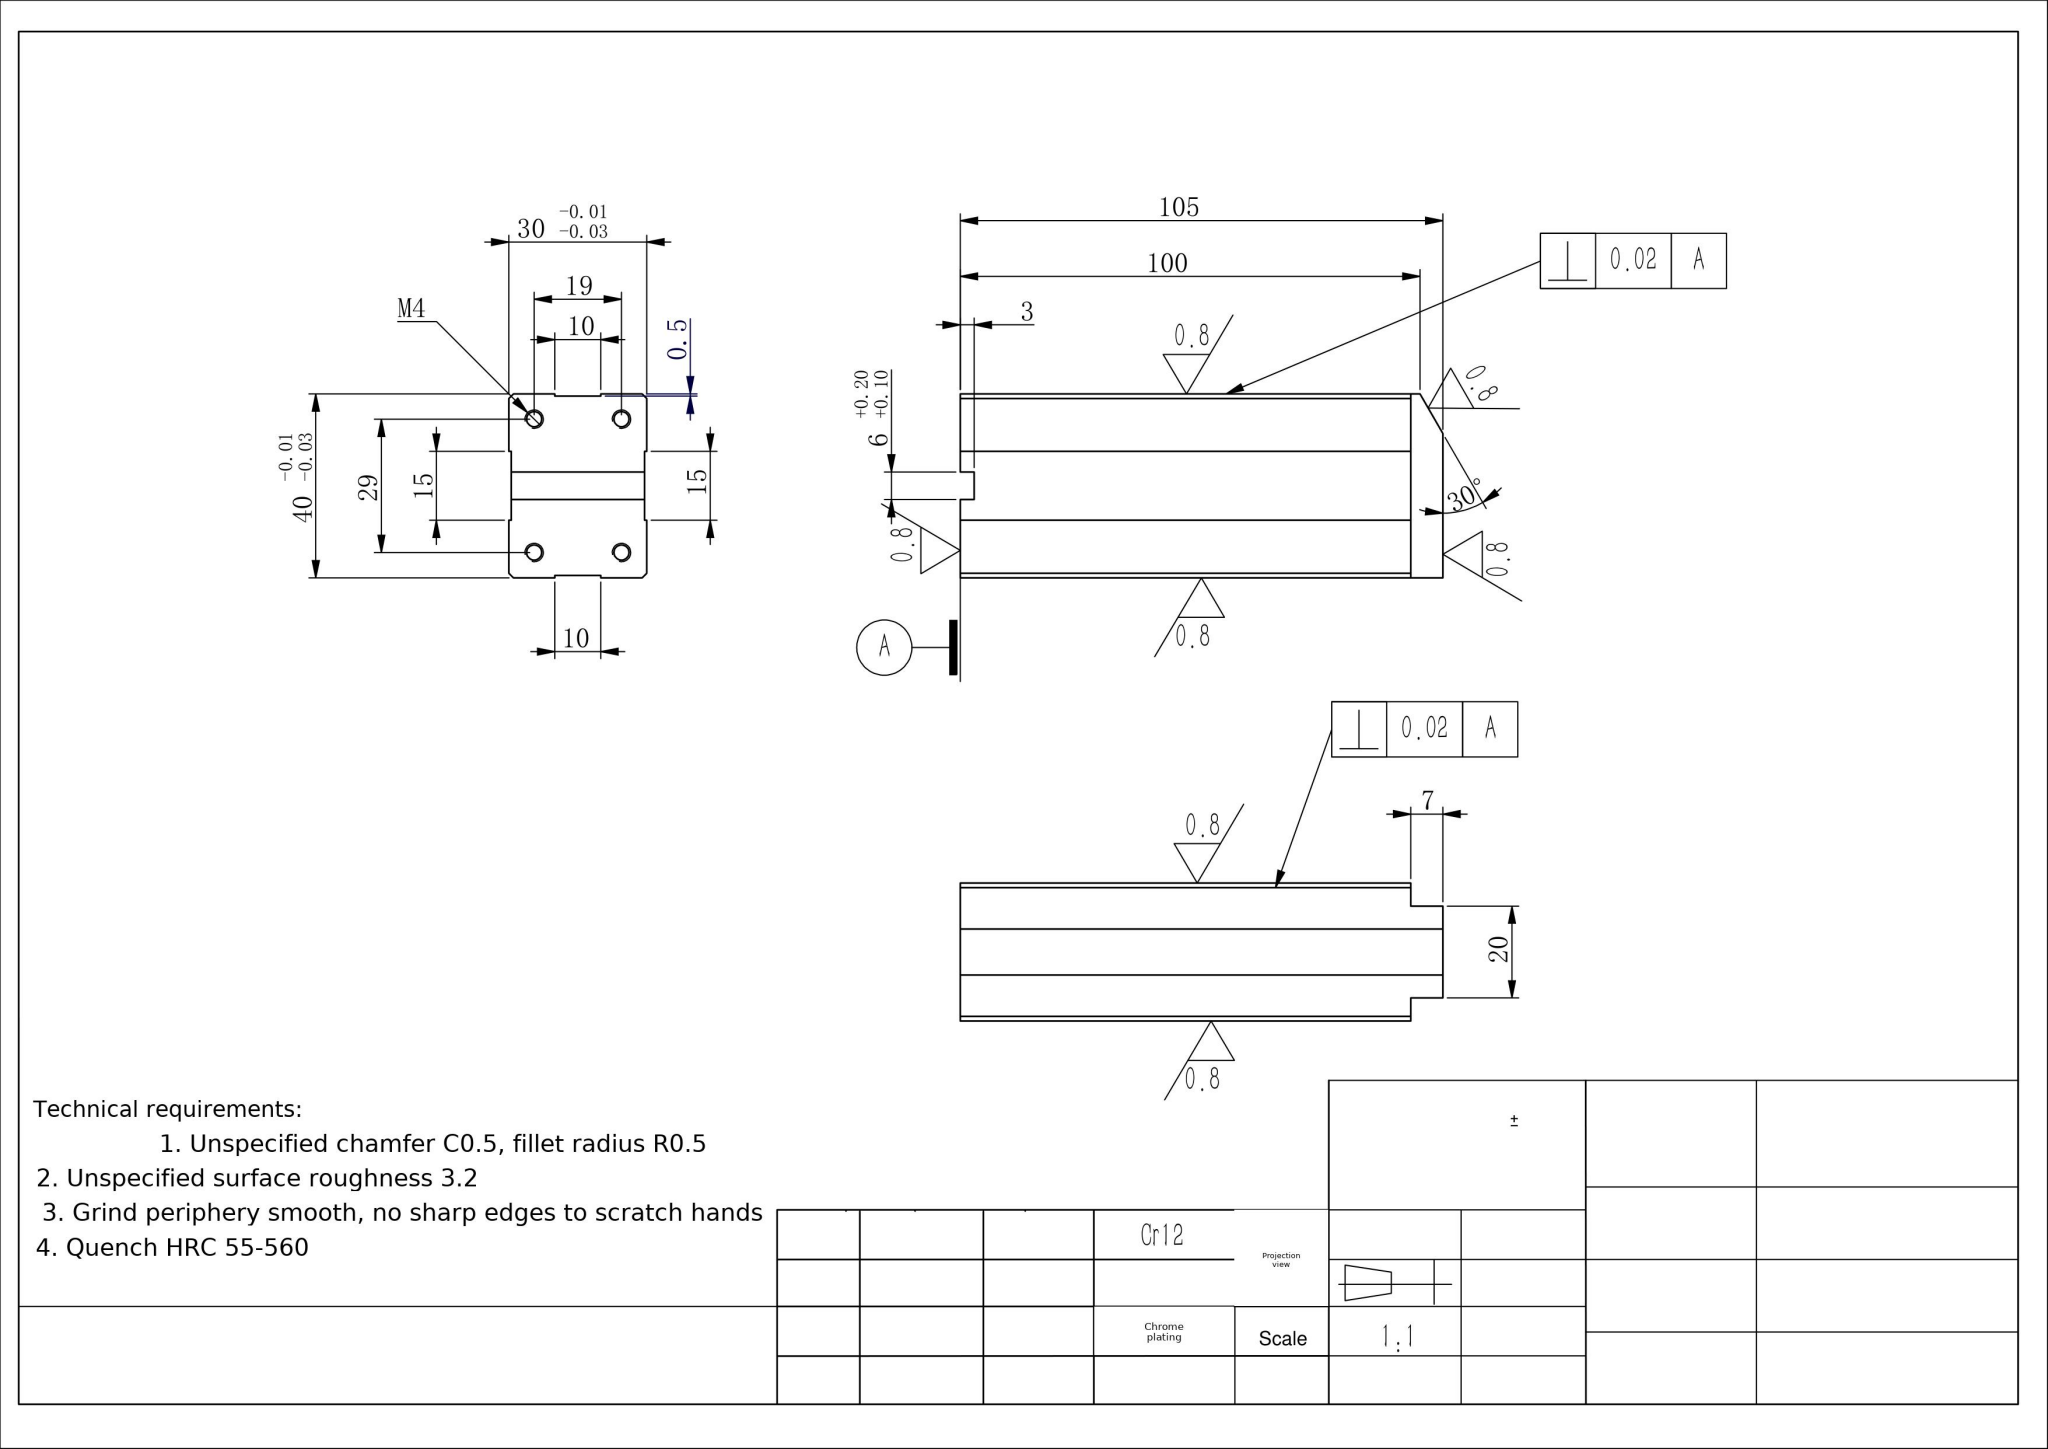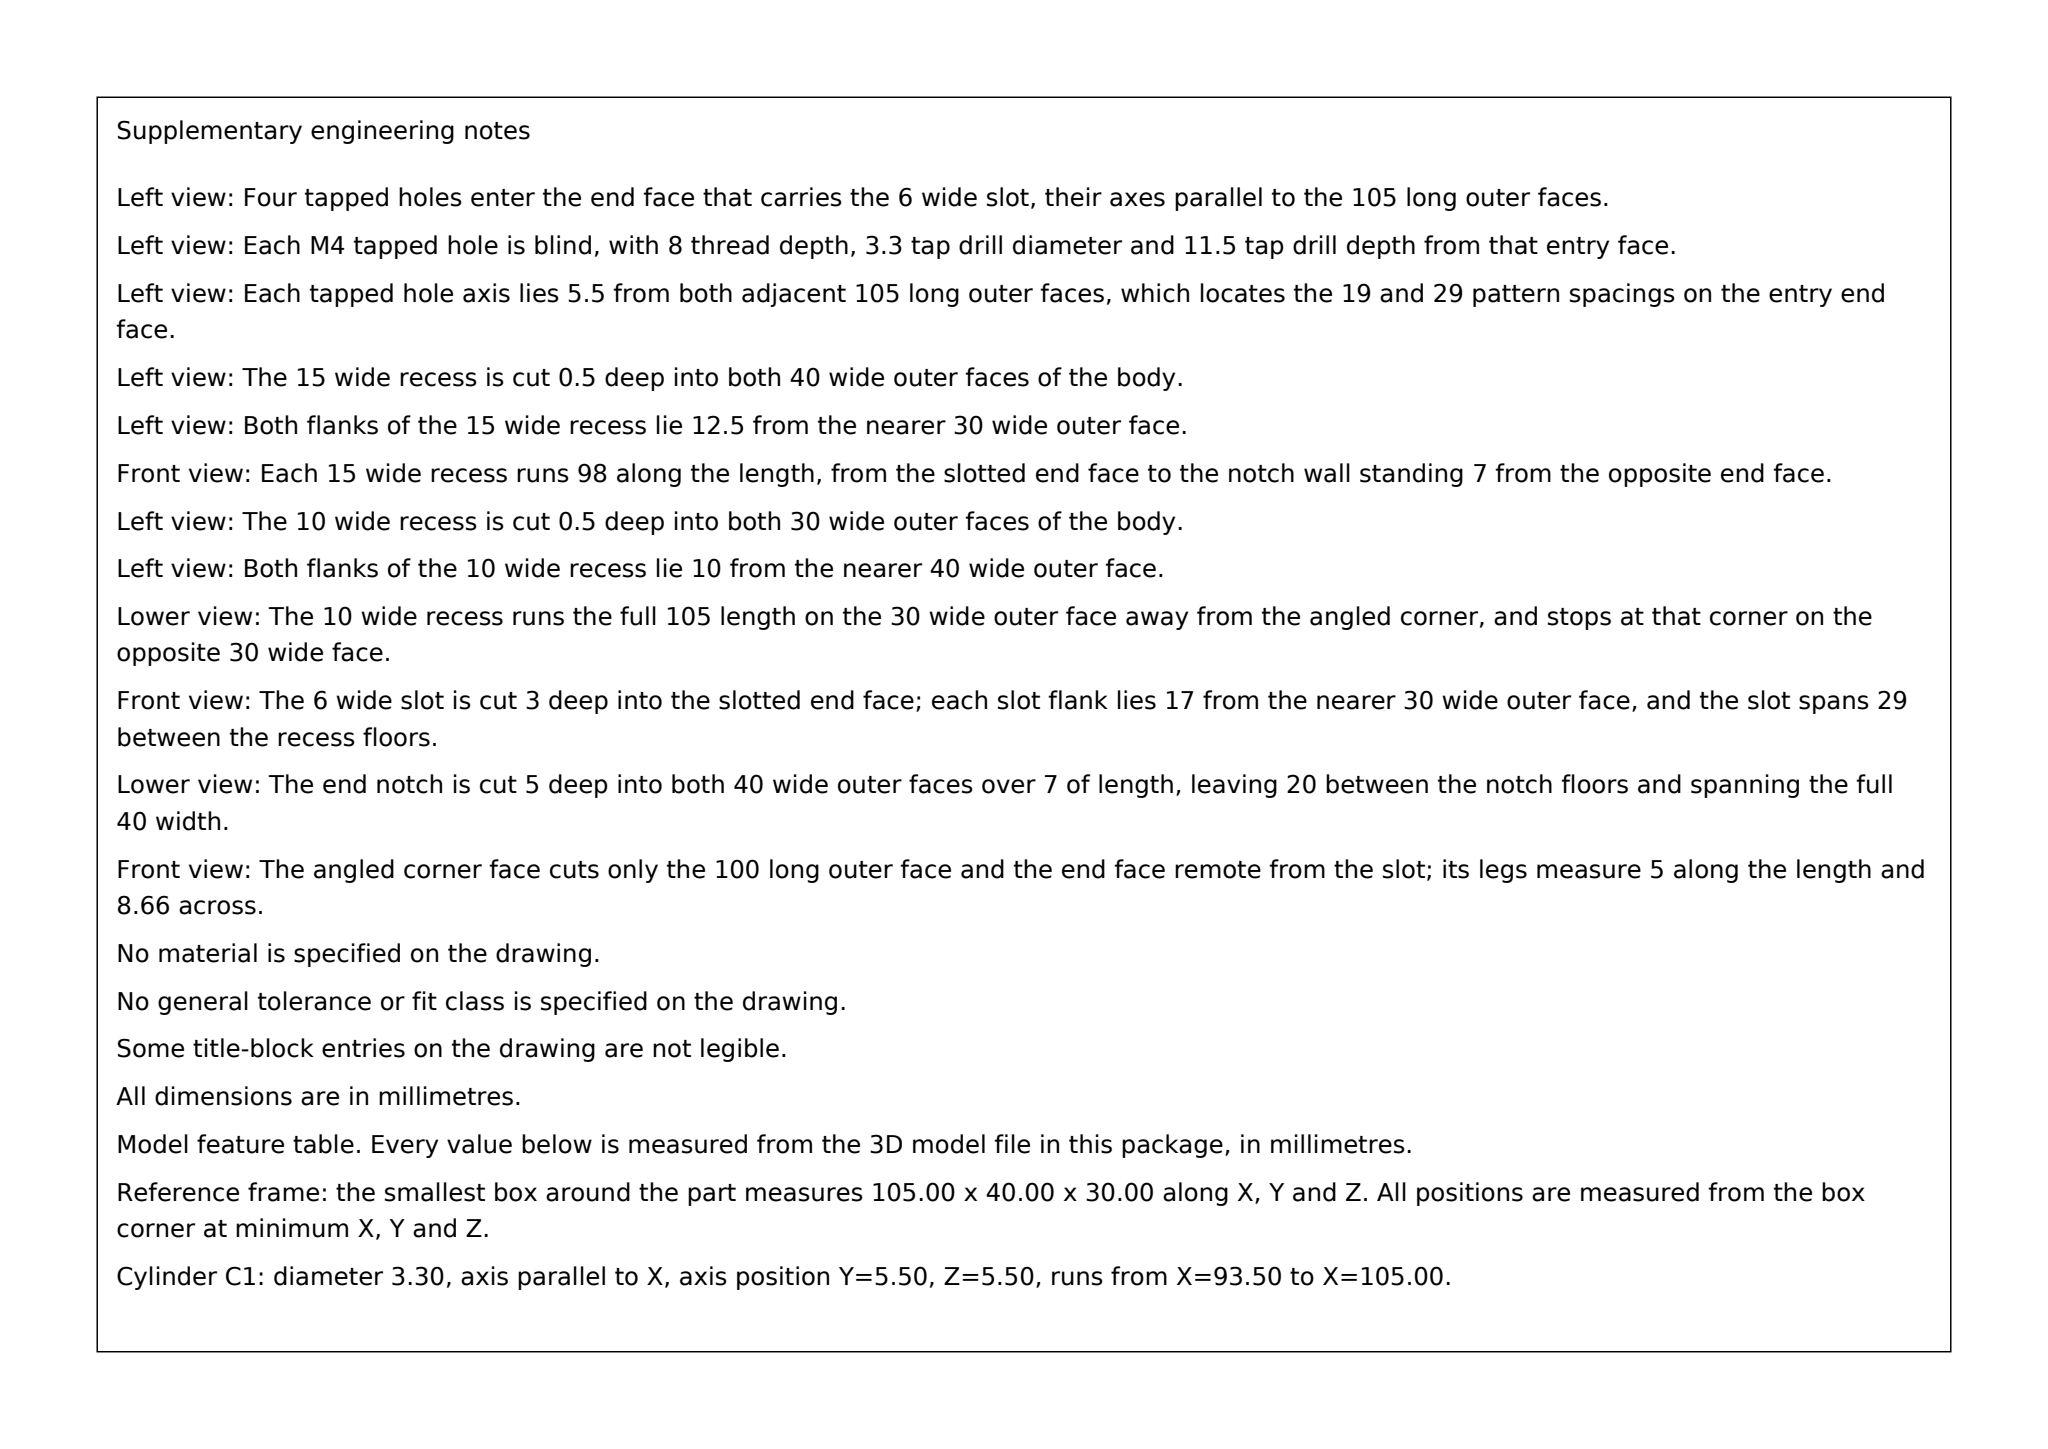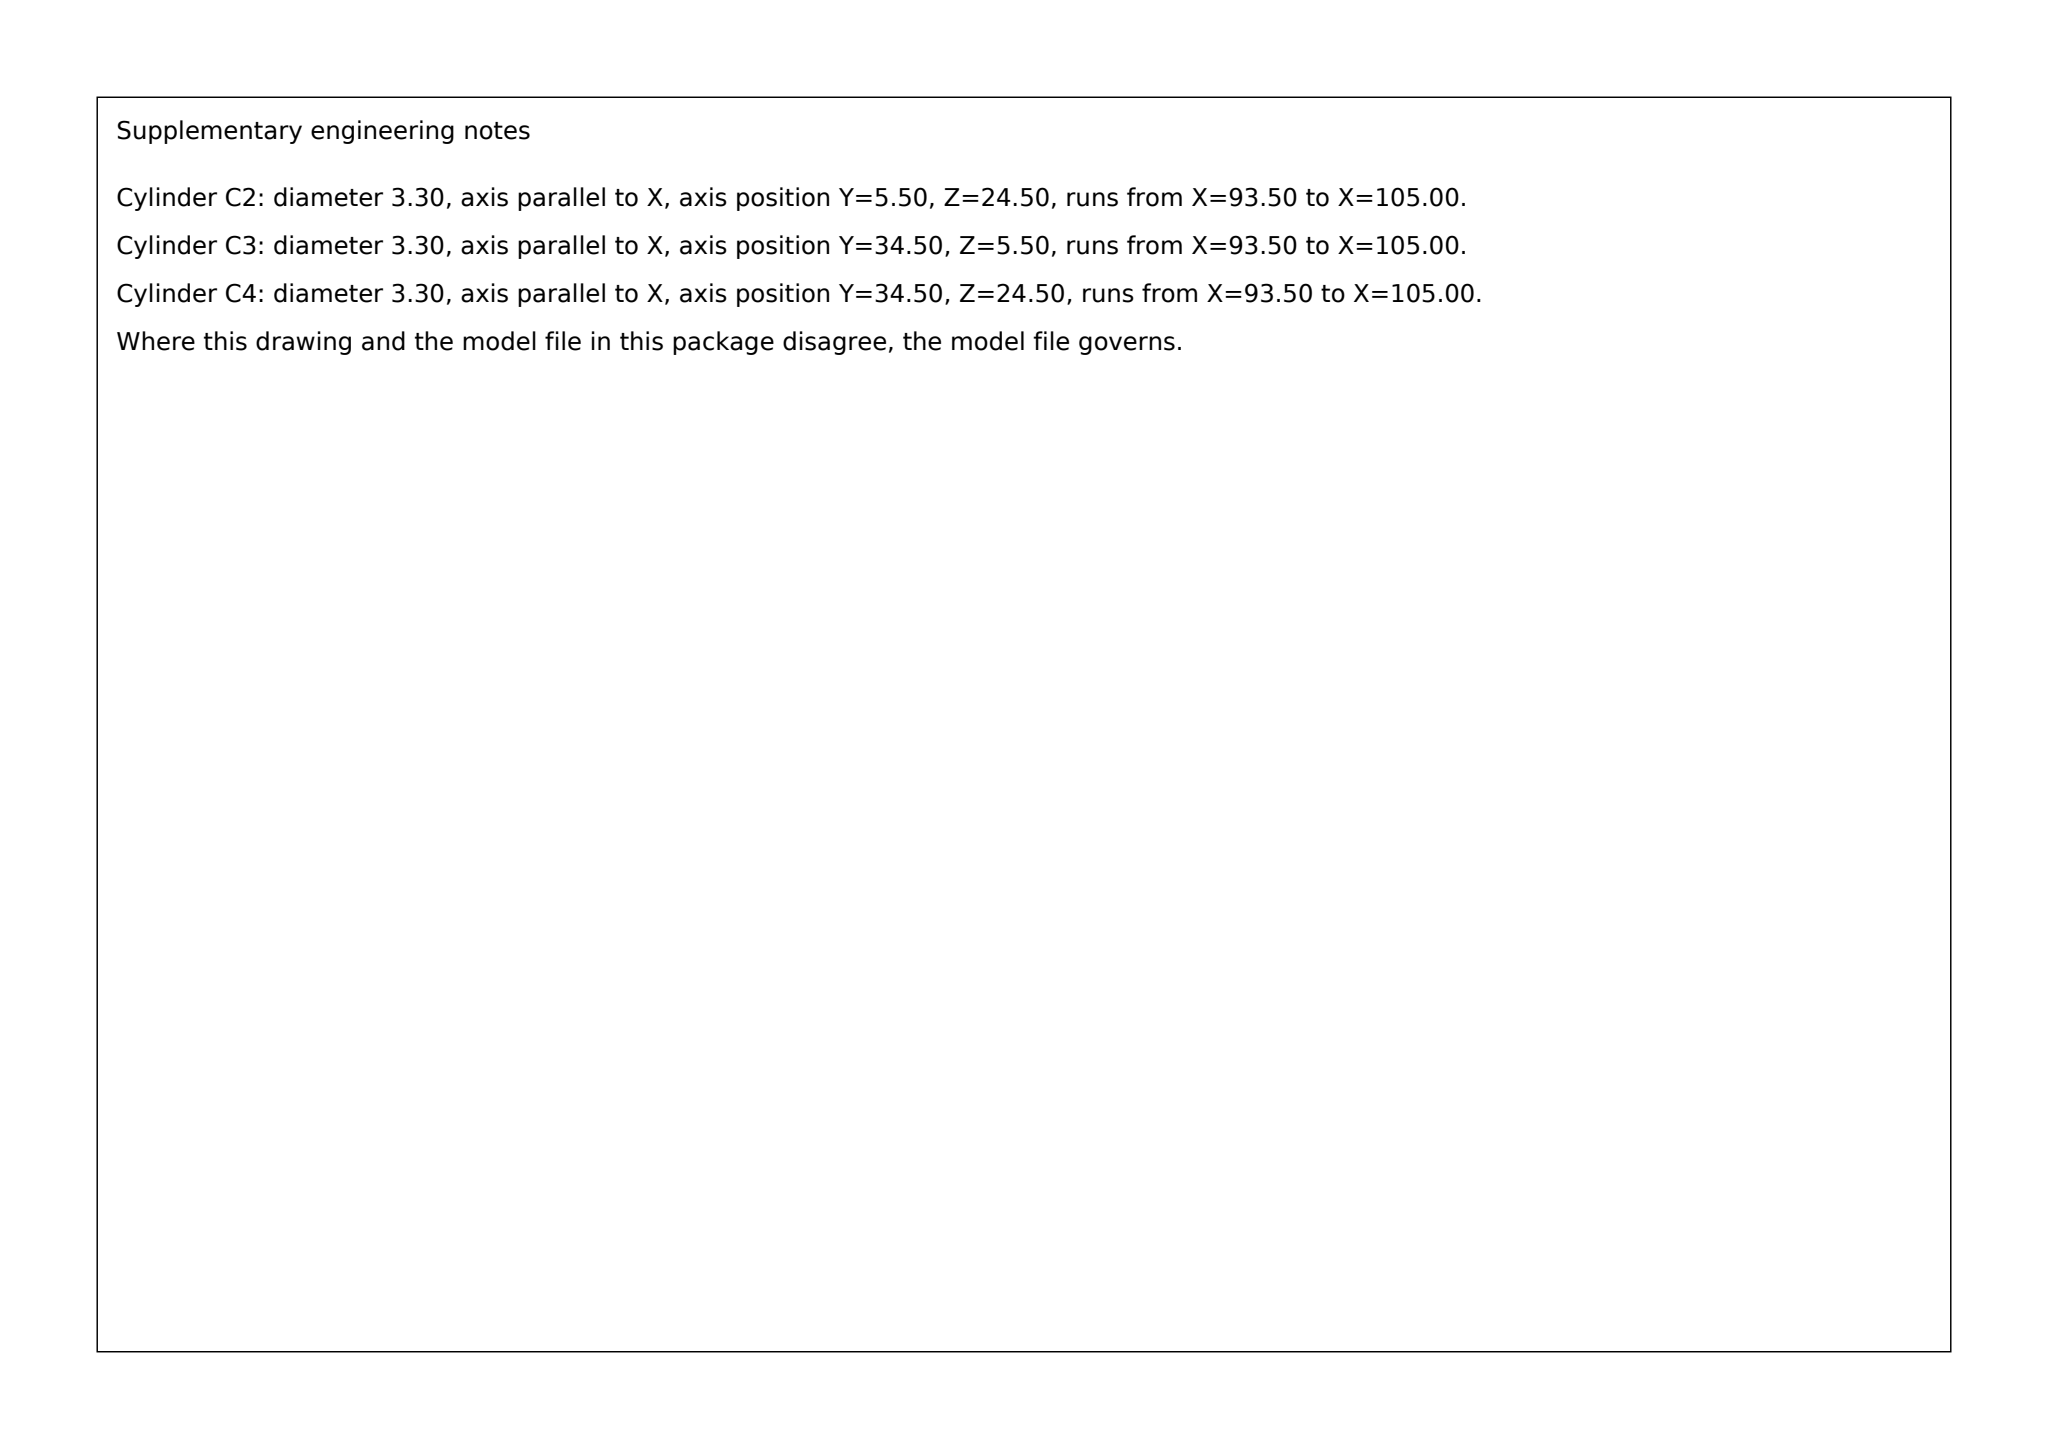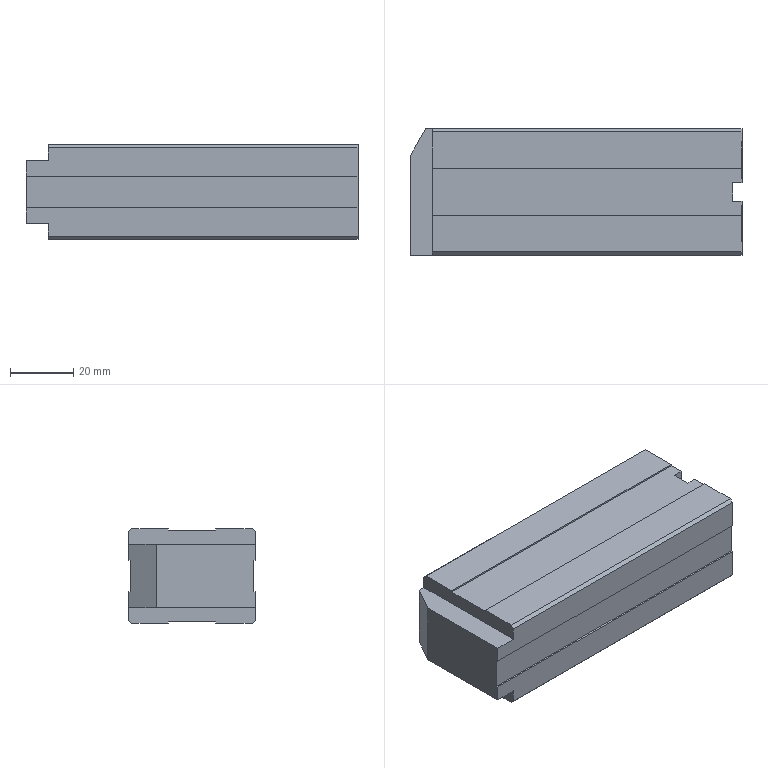Part | SolidWorks | mm | material Cr12 | 1 solid | 51 faces | box 105 x 40 x 30 mm | volume 119149 mm3 | plane 35 | cylinder 8 | cone 8 | commonest cylinder face diameters 3.3 x8